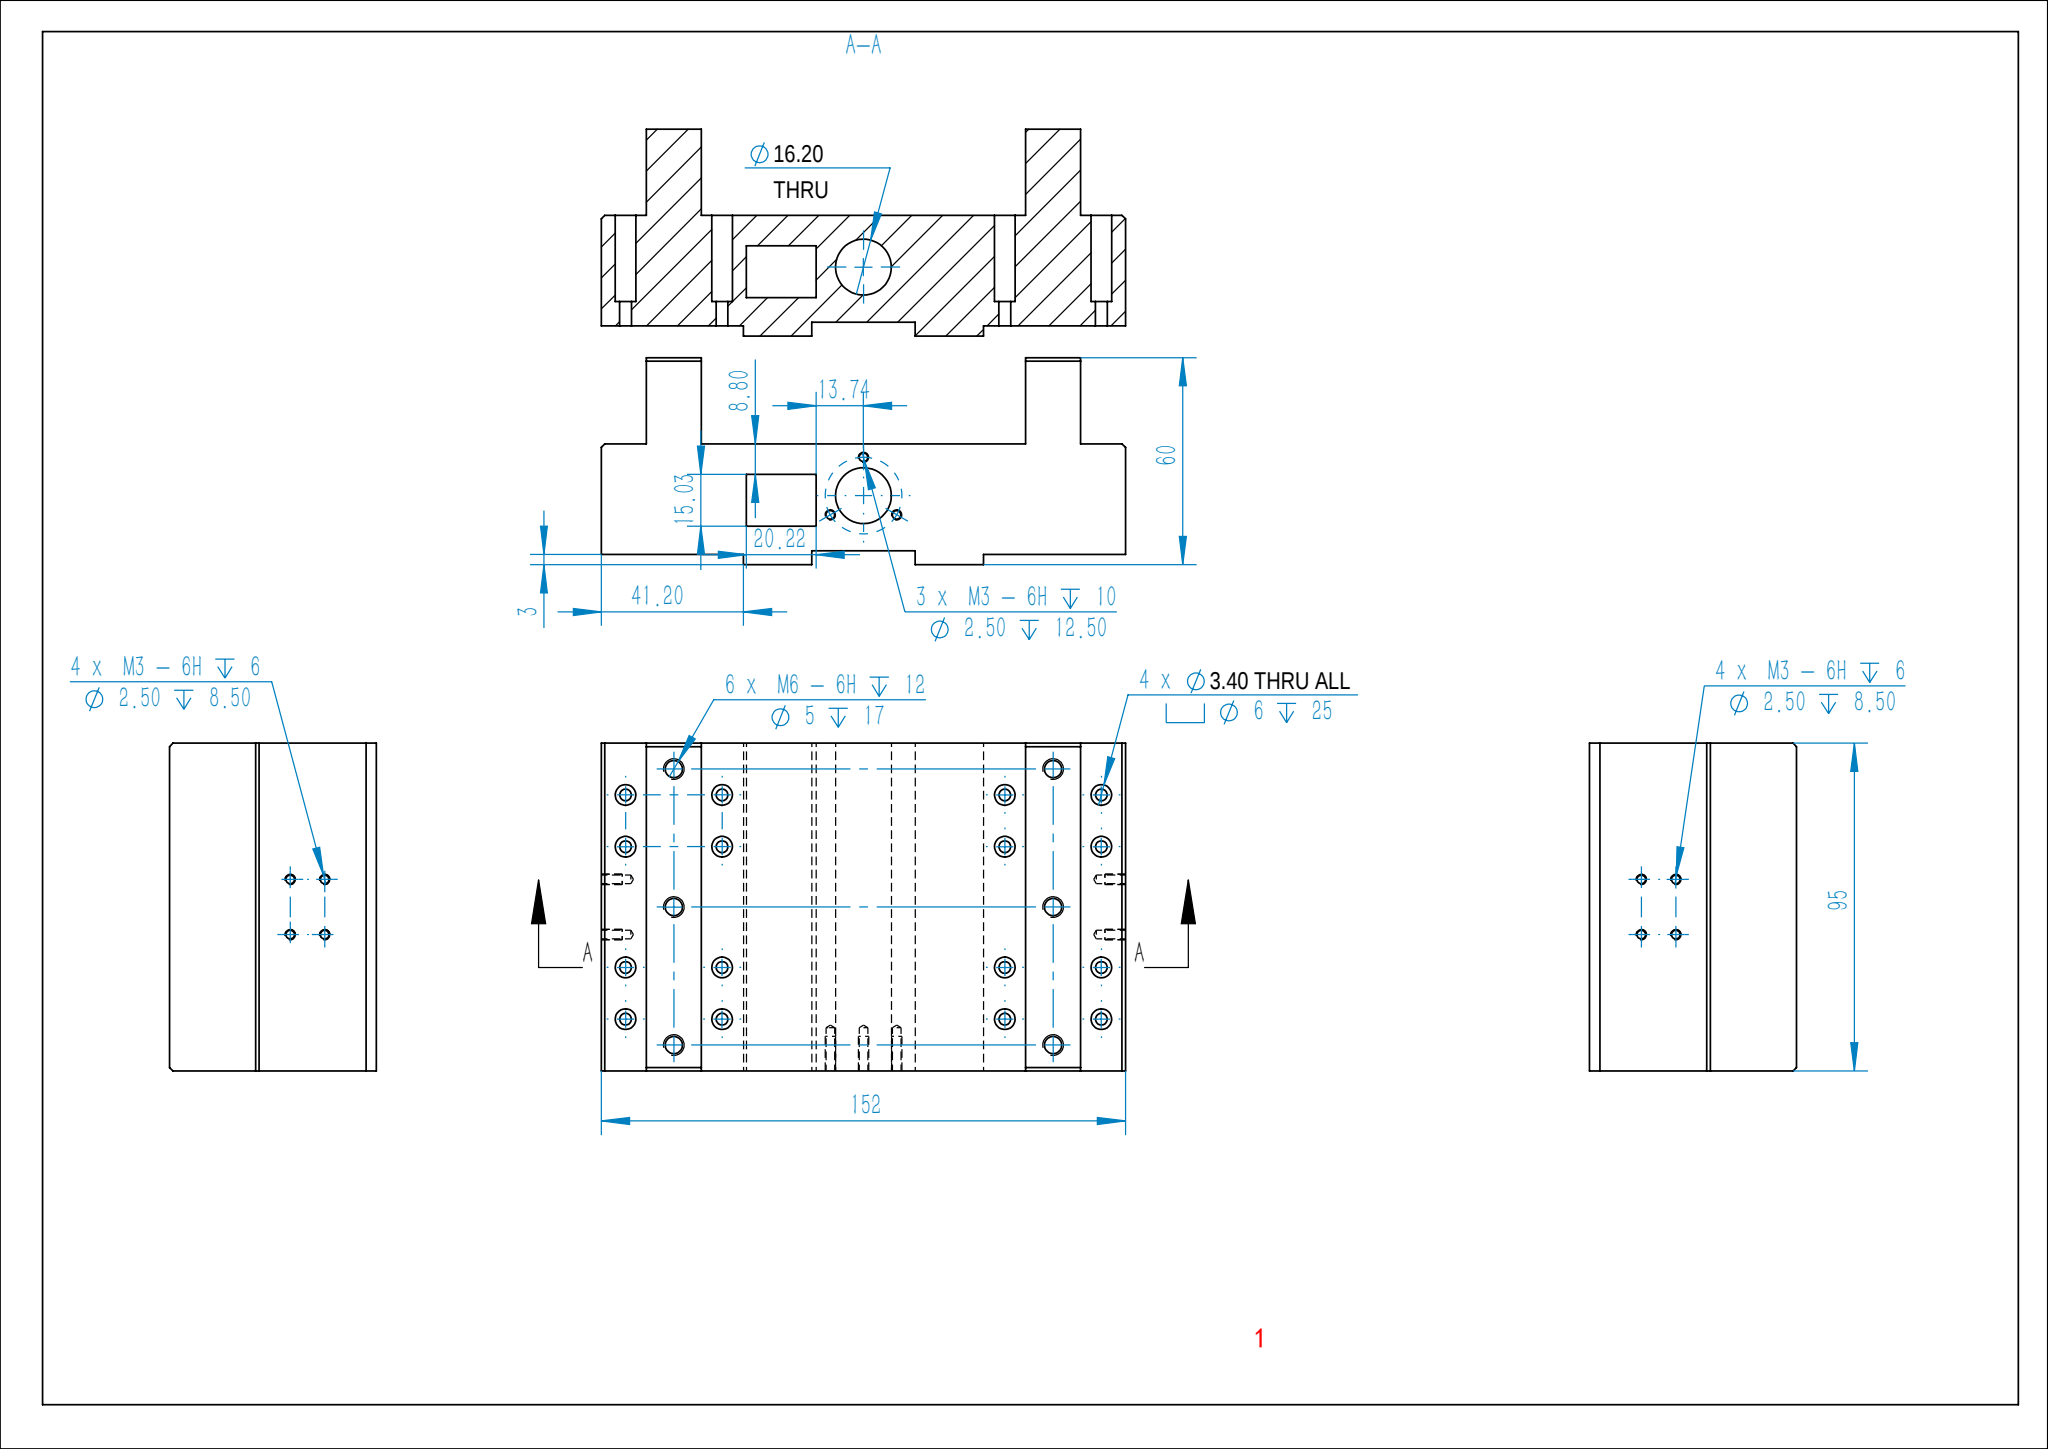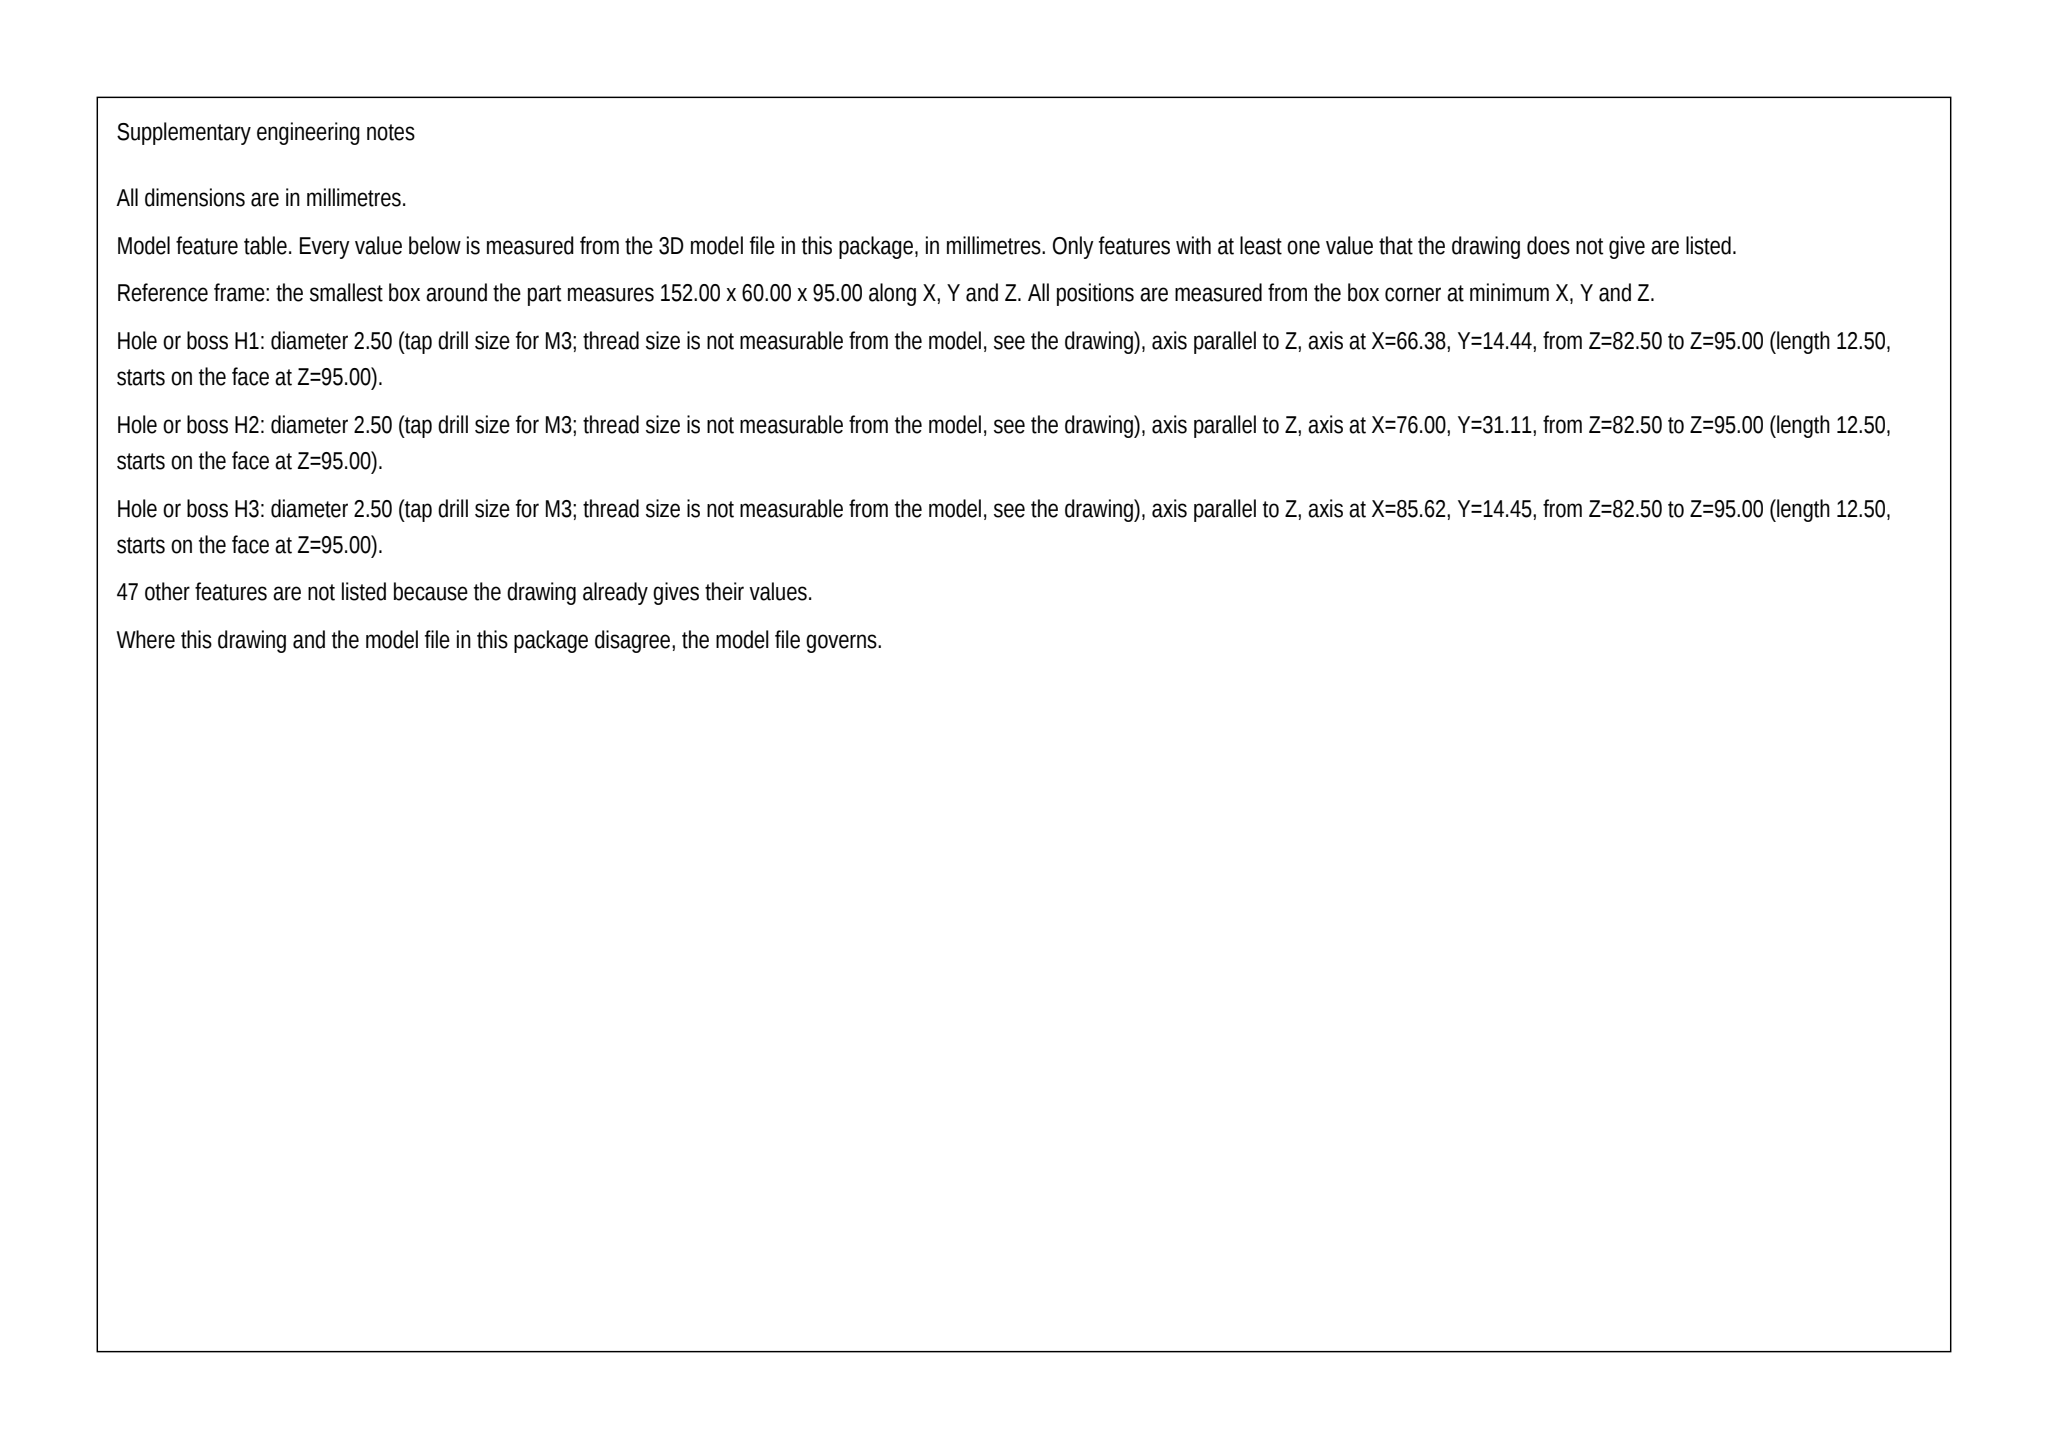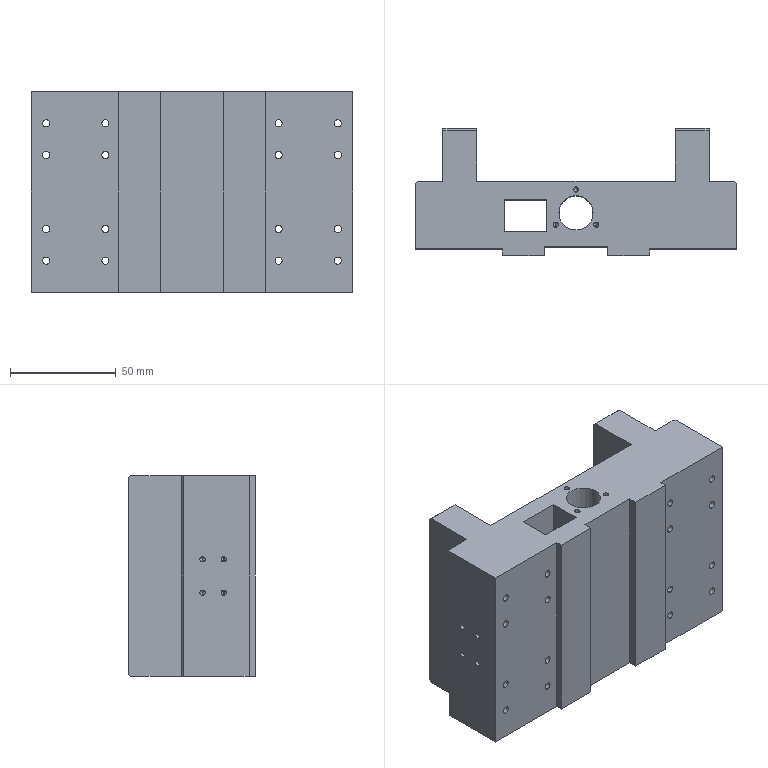Part | SolidWorks | mm | 1 solid | 182 faces | box 152 x 60 x 95 mm | volume 483023 mm3 | cylinder 100 | plane 48 | cone 34 | commonest cylinder face diameters 6 x32 3.4 x32 2.5 x22 5 x12 16.2 x2
Drawing notes:
STOCK 152 x 60 x 95 | from the solid: bbox_xyz 152 x 60 x 95
END RAILS 41.20 WIDE EA END, TOP 35 FM BASE; BOSSES 60 HIGH | from the solid: x-planes 41.2 & 110.8; y-planes 35 (rail tops), 60 (top)
END BOSSES 16 W, 13 FM EA END FACE, FULL 95 DP, Y 35 TO 60 | from the solid: x-planes 13/29 & 123/139; y 35 & y 60
BOT STEP 3 HIGH x 41.20 LG EA END, SYM ABT CL | from the solid: y-planes 0 & 3 with x-planes 41.2 / 110.8
BOT SLOT 30 W (X 61-91) SYM ABT CL x 4 HIGH FM BASE, THRU 95 | from the solid: x planes 61 & 91; y plane 4.0; no interior z-planes
RECT POCKET 20.22 W x 15.02 H THRU 95; X 42.04-62.26, Y 11.18-26.20 FM BASE | from the solid: x planes 42.04/62.26; y planes 11.18/26.20; 35-26.20=8.80
Ø16.20 BORE THRU 95, CL 76 FM EA END, 20 FM BASE | from the solid: dia 16.2 z-axis at [76.0, 20.0], length 95
3 x M3 EQ SP ON Ø22.22 B.C. ABT BORE CL, 1 AT TOP | from the solid: Ø2.5 z-holes (66.38,14.45),(76,31.11),(85.62,14.45), R=11.11 abt (76,20)
6 x M6: 2 ROWS 110 APART, 21 FM EA END; 3 @ 40 PITCH SYM ABT CL | from the solid: Ø5 y-holes x=21 & 131, z=7.5/47.5/87.5
16 x Ø3.40 THRU CBORE Ø6 DP 25: X 7 & 35 FM EA END, Z 15/30/65/80 | from the solid: Ø3.4 & Ø6 y-holes at x=7,35,117,145 by z=15,30,65,80 = 16 off
4 x M3 EA END FACE: Y 15 & 25 FM BASE, Z 39.5 & 55.5 (16 APART SYM ABT CL) | from the solid: Ø2.5 x-holes y=15/25, z=39.5/55.5, CL z=47.5
build123d program:
from build123d import *

# Parameters (mm, degrees)
SKETCH1_W                                            = 152
SKETCH1_H                                            = 60
BOSS_EXTRUDE1_DEPTH                                  = 47.5
SKETCH2_W                                            = 41.2
SKETCH2_H                                            = 3
CUT_EXTRUDE1_DEPTH                                   = 126.304
SKETCH3_R                                            = 8.1
CUT_EXTRUDE2_DEPTH                                   = 126.304
CIRPATTERN1_COUNT                                    = 3
SKETCH6_W                                            = 94
SKETCH6_H                                            = 50
CUT_EXTRUDE3_DEPTH                                   = 126.304
SKETCH7_W                                            = 13
SKETCH7_H                                            = 25
CUT_EXTRUDE4_DEPTH                                   = 126.304
LPATTERN1_COUNT                                      = 3
LPATTERN1_PITCH                                      = 40
LPATTERN1_COUNT_DIR2                                 = 2
LPATTERN1_PITCH_DIR2                                 = 110
HOLE_SIZE_ACCORDING_TO_THE_TYPE_OF_HEXAG_D           = 3.4
HOLE_SIZE_ACCORDING_TO_THE_TYPE_OF_HEXAG_CBORE_D     = 6
HOLE_SIZE_ACCORDING_TO_THE_TYPE_OF_HEXAG_CBORE_DEPTH = 25
LPATTERN2_COUNT                                      = 2
LPATTERN2_PITCH                                      = 15
LPATTERN2_COUNT_DIR2                                 = 2
LPATTERN2_PITCH_DIR2                                 = 28
MIRROR3_COPY_1_D                                     = 3.4
MIRROR3_COPY_1_CBORE_D                               = 6
MIRROR3_COPY_1_CBORE_DEPTH                           = 25
MIRROR3_COPY_2_D                                     = 3.4
MIRROR3_COPY_2_CBORE_D                               = 6
MIRROR3_COPY_2_CBORE_DEPTH                           = 25
MIRROR3_COPY_3_D                                     = 3.4
MIRROR3_COPY_3_CBORE_D                               = 6
MIRROR3_COPY_3_CBORE_DEPTH                           = 25
MIRROR4_COPY_1_D                                     = 3.4
MIRROR4_COPY_1_CBORE_D                               = 6
MIRROR4_COPY_1_CBORE_DEPTH                           = 25
MIRROR4_COPY_2_D                                     = 3.4
MIRROR4_COPY_2_CBORE_D                               = 6
MIRROR4_COPY_2_CBORE_DEPTH                           = 25
MIRROR4_COPY_3_D                                     = 3.4
MIRROR4_COPY_3_CBORE_D                               = 6
MIRROR4_COPY_3_CBORE_DEPTH                           = 25
MIRROR4_COPY_4_D                                     = 3.4
MIRROR4_COPY_4_CBORE_D                               = 6
MIRROR4_COPY_4_CBORE_DEPTH                           = 25
MIRROR4_COPY_5_D                                     = 3.4
MIRROR4_COPY_5_CBORE_D                               = 6
MIRROR4_COPY_5_CBORE_DEPTH                           = 25
MIRROR4_COPY_6_D                                     = 3.4
MIRROR4_COPY_6_CBORE_D                               = 6
MIRROR4_COPY_6_CBORE_DEPTH                           = 25
MIRROR4_COPY_7_D                                     = 3.4
MIRROR4_COPY_7_CBORE_D                               = 6
MIRROR4_COPY_7_CBORE_DEPTH                           = 25
CHAMFER1_SIZE                                        = 1
CHAMFER2_SIZE                                        = 1
LPATTERN3_COUNT                                      = 2
LPATTERN3_PITCH                                      = 10
LPATTERN3_COUNT_DIR2                                 = 2
LPATTERN3_PITCH_DIR2                                 = 16
SKETCH15_W                                           = 30
SKETCH15_H                                           = 8
CUT_EXTRUDE5_DEPTH                                   = 126.304
SKETCH17_W                                           = 20.217
SKETCH17_H                                           = 15.029
CUT_EXTRUDE7_DEPTH                                   = 163


with BuildPart() as part:
    # Sketch1 → Boss-Extrude1 (new, symmetric)
    with BuildSketch(Plane.XY):
        Rectangle(SKETCH1_W, SKETCH1_H)
    extrude(amount=BOSS_EXTRUDE1_DEPTH, both=True)

    # Sketch2 → Cut-Extrude1 (cut, through all)
    with BuildSketch(Plane.XY.offset(47.5)):
        with Locations((-55.4, -28.5)):
            Rectangle(SKETCH2_W, SKETCH2_H)
    cut_extrude1 = extrude(amount=-CUT_EXTRUDE1_DEPTH, mode=Mode.SUBTRACT)

    # Mirror1: Cut-Extrude1 across plane
    add(cut_extrude1.mirror(Plane(origin=(0, 0, 0), x_dir=(0, 0, 1), z_dir=(1, 0, 0))), mode=Mode.SUBTRACT)

    # Sketch3 → Cut-Extrude2 (cut, through all)
    with BuildSketch(Plane.XY.offset(47.5)):
        with Locations((0, -10)):
            Circle(SKETCH3_R)
    extrude(amount=-CUT_EXTRUDE2_DEPTH, mode=Mode.SUBTRACT)

    # Sketch4 → M3 Tapped Hole1 (revolve, cut)
    with BuildSketch(Plane(origin=(0, 1.11, 47.5), x_dir=(0, -1, 0), z_dir=(1, 0, 0))):
        Polygon((0, 0), (0, 13.251), (1.25, 12.5), (1.25, 0), align=None)
    m3_tapped_hole1 = revolve(axis=Axis((0, 1.11, 53.85), (0, 0, -1)), mode=Mode.SUBTRACT)

    # CirPattern1: M3 Tapped Hole1 ×3 about axis
    cirpattern1_axis = Axis((0, -10, 0), (0, 0, 1))
    for i in range(1, CIRPATTERN1_COUNT):
        add(m3_tapped_hole1.rotate(cirpattern1_axis, i * 360 / CIRPATTERN1_COUNT), mode=Mode.SUBTRACT)

    # Sketch6 → Cut-Extrude3 (cut, through all)
    with BuildSketch(Plane.XY.offset(47.5)):
        with Locations((0, 30)):
            Rectangle(SKETCH6_W, SKETCH6_H)
    extrude(amount=-CUT_EXTRUDE3_DEPTH, mode=Mode.SUBTRACT)

    # Sketch7 → Cut-Extrude4 (cut, through all)
    with BuildSketch(Plane.XY.offset(47.5)):
        with Locations((-69.5, 17.5)):
            Rectangle(SKETCH7_W, SKETCH7_H)
    cut_extrude4 = extrude(amount=-CUT_EXTRUDE4_DEPTH, mode=Mode.SUBTRACT)

    # Mirror2: Cut-Extrude4 across plane
    add(cut_extrude4.mirror(Plane(origin=(0, 0, 0), x_dir=(0, 0, 1), z_dir=(1, 0, 0))), mode=Mode.SUBTRACT)

    # Sketch8 → M6 Tapped Hole1 (revolve, cut)
    with BuildSketch(Plane(origin=(-55, 30, -40), x_dir=(0, 0, 1), z_dir=(1, 0, 0))):
        Polygon((0, 0), (0, 18.502), (2.5, 17), (2.5, 0), align=None)
    m6_tapped_hole1 = revolve(axis=Axis((-55, 36.35, -40), (0, -1, 0)), mode=Mode.SUBTRACT)

    # LPattern1: M6 Tapped Hole1 3 × 2
    with Locations(*[(j * LPATTERN1_PITCH_DIR2, 0, i * LPATTERN1_PITCH) for i in range(LPATTERN1_COUNT) for j in range(LPATTERN1_COUNT_DIR2) if (i, j) != (0, 0)]):
        add(m6_tapped_hole1, mode=Mode.SUBTRACT)

    # Hole size according to the type of hexag (through all)
    with Locations(Plane(origin=(0, 5, 0), x_dir=(1, 0, 0), z_dir=(0, 1, 0))):
        with Locations((-69, 32.5)):
            hole_size_according_to_the_type_of_hexag = CounterBoreHole(HOLE_SIZE_ACCORDING_TO_THE_TYPE_OF_HEXAG_D / 2, HOLE_SIZE_ACCORDING_TO_THE_TYPE_OF_HEXAG_CBORE_D / 2, HOLE_SIZE_ACCORDING_TO_THE_TYPE_OF_HEXAG_CBORE_DEPTH)

    # LPattern2: Hole size according to the type of hexag 2 × 2
    with Locations(*[(j * LPATTERN2_PITCH_DIR2, 0, i * LPATTERN2_PITCH) for i in range(LPATTERN2_COUNT) for j in range(LPATTERN2_COUNT_DIR2) if (i, j) != (0, 0)]):
        add(hole_size_according_to_the_type_of_hexag, mode=Mode.SUBTRACT)

    # Mirror3: Hole size according to the type of hexag across plane
    add(hole_size_according_to_the_type_of_hexag.mirror(Plane(origin=(0, 0, 0), x_dir=(0, 0, 1), z_dir=(1, 0, 0))), mode=Mode.SUBTRACT)

    # Mirror3 copy 1 (through all)
    with Locations(Plane(origin=(-28, 5, 0), x_dir=(-1, 0, 0), z_dir=(0, 1, 0))):
        with Locations((-69, -32.5)):
            CounterBoreHole(MIRROR3_COPY_1_D / 2, MIRROR3_COPY_1_CBORE_D / 2, MIRROR3_COPY_1_CBORE_DEPTH)

    # Mirror3 copy 2 (through all)
    with Locations(Plane(origin=(0, 5, 15), x_dir=(-1, 0, 0), z_dir=(0, 1, 0))):
        with Locations((-69, -32.5)):
            CounterBoreHole(MIRROR3_COPY_2_D / 2, MIRROR3_COPY_2_CBORE_D / 2, MIRROR3_COPY_2_CBORE_DEPTH)

    # Mirror3 copy 3 (through all)
    with Locations(Plane(origin=(-28, 5, 15), x_dir=(-1, 0, 0), z_dir=(0, 1, 0))):
        with Locations((-69, -32.5)):
            CounterBoreHole(MIRROR3_COPY_3_D / 2, MIRROR3_COPY_3_CBORE_D / 2, MIRROR3_COPY_3_CBORE_DEPTH)

    # Mirror4: Hole size according to the type of hexag across plane
    add(hole_size_according_to_the_type_of_hexag.mirror(Plane.XY), mode=Mode.SUBTRACT)

    # Mirror4 copy 1 (through all)
    with Locations(Plane(origin=(28, 5, 0), x_dir=(1, 0, 0), z_dir=(0, 1, 0))):
        with Locations((-69, -32.5)):
            CounterBoreHole(MIRROR4_COPY_1_D / 2, MIRROR4_COPY_1_CBORE_D / 2, MIRROR4_COPY_1_CBORE_DEPTH)

    # Mirror4 copy 2 (through all)
    with Locations(Plane(origin=(0, 5, -15), x_dir=(1, 0, 0), z_dir=(0, 1, 0))):
        with Locations((-69, -32.5)):
            CounterBoreHole(MIRROR4_COPY_2_D / 2, MIRROR4_COPY_2_CBORE_D / 2, MIRROR4_COPY_2_CBORE_DEPTH)

    # Mirror4 copy 3 (through all)
    with Locations(Plane(origin=(28, 5, -15), x_dir=(1, 0, 0), z_dir=(0, 1, 0))):
        with Locations((-69, -32.5)):
            CounterBoreHole(MIRROR4_COPY_3_D / 2, MIRROR4_COPY_3_CBORE_D / 2, MIRROR4_COPY_3_CBORE_DEPTH)

    # Mirror4 copy 4 (through all)
    with Locations(Plane(origin=(0, 5, 0), x_dir=(-1, 0, 0), z_dir=(0, 1, 0))):
        with Locations((-69, 32.5)):
            CounterBoreHole(MIRROR4_COPY_4_D / 2, MIRROR4_COPY_4_CBORE_D / 2, MIRROR4_COPY_4_CBORE_DEPTH)

    # Mirror4 copy 5 (through all)
    with Locations(Plane(origin=(-28, 5, 0), x_dir=(-1, 0, 0), z_dir=(0, 1, 0))):
        with Locations((-69, 32.5)):
            CounterBoreHole(MIRROR4_COPY_5_D / 2, MIRROR4_COPY_5_CBORE_D / 2, MIRROR4_COPY_5_CBORE_DEPTH)

    # Mirror4 copy 6 (through all)
    with Locations(Plane(origin=(0, 5, -15), x_dir=(-1, 0, 0), z_dir=(0, 1, 0))):
        with Locations((-69, 32.5)):
            CounterBoreHole(MIRROR4_COPY_6_D / 2, MIRROR4_COPY_6_CBORE_D / 2, MIRROR4_COPY_6_CBORE_DEPTH)

    # Mirror4 copy 7 (through all)
    with Locations(Plane(origin=(-28, 5, -15), x_dir=(-1, 0, 0), z_dir=(0, 1, 0))):
        with Locations((-69, 32.5)):
            CounterBoreHole(MIRROR4_COPY_7_D / 2, MIRROR4_COPY_7_CBORE_D / 2, MIRROR4_COPY_7_CBORE_DEPTH)

    # Chamfer1
    chamfer1_edges = [part.edges().sort_by_distance(p)[0] for p in [
        (-55, 30, -47.5),
        (-55, 30, 47.5),
        (55, 30, -47.5),
        (55, 30, 47.5),
    ]]
    chamfer(chamfer1_edges, length=CHAMFER1_SIZE)

    # Chamfer2
    chamfer2_edges = [part.edges().sort_by_distance(p)[0] for p in [
        (76, 5, 0),
        (-76, 5, 0),
    ]]
    chamfer(chamfer2_edges, length=CHAMFER2_SIZE)

    # Sketch12 → M3 Tapped Hole2 (revolve, cut)
    with BuildSketch(Plane(origin=(76, -15, -8), x_dir=(0, 0, -1), z_dir=(0, 1, 0))):
        Polygon((0, 0), (0, 9.251), (1.25, 8.5), (1.25, 0), align=None)
    m3_tapped_hole2 = revolve(axis=Axis((82.35, -15, -8), (-1, 0, 0)), mode=Mode.SUBTRACT)

    # LPattern3: M3 Tapped Hole2 2 × 2
    with Locations(*[(0, i * LPATTERN3_PITCH, j * LPATTERN3_PITCH_DIR2) for i in range(LPATTERN3_COUNT) for j in range(LPATTERN3_COUNT_DIR2) if (i, j) != (0, 0)]):
        add(m3_tapped_hole2, mode=Mode.SUBTRACT)

    # Mirror5: M3 Tapped Hole2 across plane
    add(m3_tapped_hole2.mirror(Plane(origin=(0, 0, 0), x_dir=(0, 0, 1), z_dir=(1, 0, 0))), mode=Mode.SUBTRACT)

    # Mirror5 copy 1 sketch → Mirror5 copy 1 (revolve, cut)
    with BuildSketch(Plane(origin=(-76, -15, 8), x_dir=(0, 0, -1), z_dir=(0, 1, 0))):
        Polygon((0, 0), (0, -9.251), (1.25, -8.5), (1.25, 0), align=None)
    revolve(axis=Axis((-82.35, -15, 8), (-1, 0, 0)), mode=Mode.SUBTRACT)

    # Mirror5 copy 2 sketch → Mirror5 copy 2 (revolve, cut)
    with BuildSketch(Plane(origin=(-76, -5, -8), x_dir=(0, 0, -1), z_dir=(0, 1, 0))):
        Polygon((0, 0), (0, -9.251), (1.25, -8.5), (1.25, 0), align=None)
    revolve(axis=Axis((-82.35, -5, -8), (-1, 0, 0)), mode=Mode.SUBTRACT)

    # Mirror5 copy 3 sketch → Mirror5 copy 3 (revolve, cut)
    with BuildSketch(Plane(origin=(-76, -5, 8), x_dir=(0, 0, -1), z_dir=(0, 1, 0))):
        Polygon((0, 0), (0, -9.251), (1.25, -8.5), (1.25, 0), align=None)
    revolve(axis=Axis((-82.35, -5, 8), (-1, 0, 0)), mode=Mode.SUBTRACT)

    # Sketch15 → Cut-Extrude5 (cut, through all)
    with BuildSketch(Plane.XY.offset(47.5)):
        with Locations((0, -30)):
            Rectangle(SKETCH15_W, SKETCH15_H)
    extrude(amount=-CUT_EXTRUDE5_DEPTH, mode=Mode.SUBTRACT)

    # Sketch17 → Cut-Extrude7 (cut)
    with BuildSketch(Plane(origin=(0, 0, -47.5), x_dir=(-1, 0, 0), z_dir=(0, 0, -1))):
        with Locations((23.851, -11.31)):
            Rectangle(SKETCH17_W, SKETCH17_H)
    extrude(amount=-CUT_EXTRUDE7_DEPTH, mode=Mode.SUBTRACT)


solid = part.part